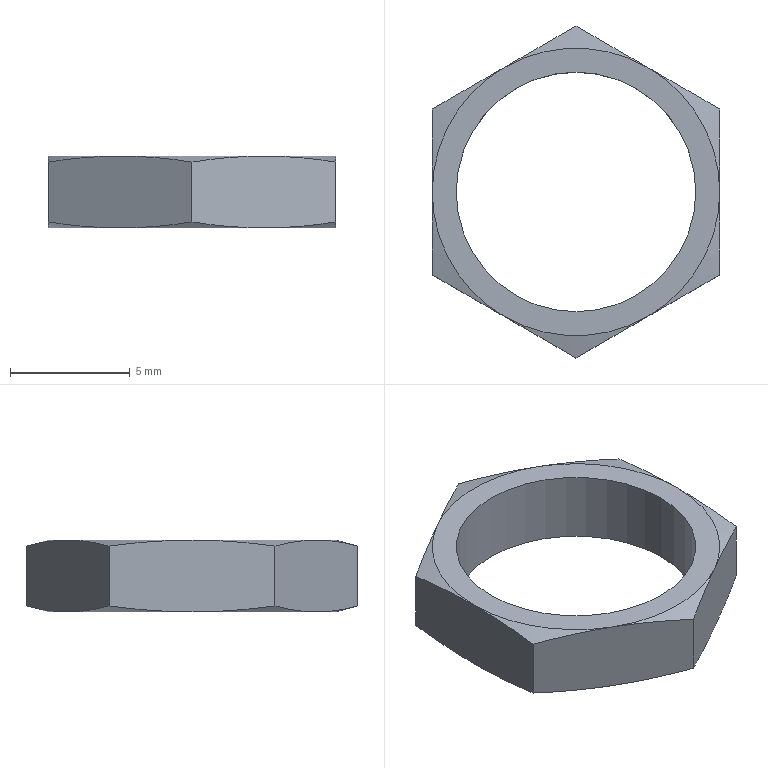Component | SolidWorks | gbgbCJPB6-5-B(0)F8-1_gbgbSNPS-006_CJPF8-2 | 1 solid | 22 faces | box 12 x 13.86 x 3 mm | volume 137 mm3 | cone 12 | plane 8 | cylinder 2 | commonest cylinder face diameters 10 x2
STEP:
#1=COLOUR_RGB('',0.7922,0.8196,0.9333);
#2=FILL_AREA_STYLE_COLOUR('',#1);
#3=FILL_AREA_STYLE('',(#2));
#4=SURFACE_STYLE_FILL_AREA(#3);
#5=SURFACE_SIDE_STYLE('',(#4));
#6=SURFACE_STYLE_USAGE(.BOTH.,#5);
#7=PRESENTATION_STYLE_ASSIGNMENT((#6));
#8=CARTESIAN_POINT('',(2.212,14.172,15.836));
#9=VERTEX_POINT('',#8);
#10=CARTESIAN_POINT('',(2.606,14.172,15.836));
#11=VERTEX_POINT('',#10);
#12=CARTESIAN_POINT('',(2.409,14.172,15.836));
#13=DIRECTION('',(0.,0.,1.));
#14=DIRECTION('',(-1.,0.,0.));
#15=AXIS2_PLACEMENT_3D('',#12,#13,#14);
#16=CIRCLE('',#15,0.1969);
#17=EDGE_CURVE('',#9,#11,#16,.T.);
#18=ORIENTED_EDGE('',*,*,#17,.F.);
#19=CARTESIAN_POINT('',(2.212,14.172,15.954));
#20=VERTEX_POINT('',#19);
#21=CARTESIAN_POINT('',(2.212,14.172,15.836));
#22=DIRECTION('',(0.,0.,1.));
#23=VECTOR('',#22,39.37);
#24=LINE('',#21,#23);
#25=EDGE_CURVE('',#9,#20,#24,.T.);
#26=ORIENTED_EDGE('',*,*,#25,.T.);
#27=CARTESIAN_POINT('',(2.606,14.172,15.954));
#28=VERTEX_POINT('',#27);
#29=CARTESIAN_POINT('',(2.409,14.172,15.954));
#30=DIRECTION('',(0.,0.,1.));
#31=DIRECTION('',(1.,0.,0.));
#32=AXIS2_PLACEMENT_3D('',#29,#30,#31);
#33=CIRCLE('',#32,0.1969);
#34=EDGE_CURVE('',#20,#28,#33,.T.);
#35=ORIENTED_EDGE('',*,*,#34,.T.);
#36=CARTESIAN_POINT('',(2.606,14.172,15.836));
#37=DIRECTION('',(0.,0.,1.));
#38=VECTOR('',#37,39.37);
#39=LINE('',#36,#38);
#40=EDGE_CURVE('',#11,#28,#39,.T.);
#41=ORIENTED_EDGE('',*,*,#40,.F.);
#42=EDGE_LOOP('',(#18,#26,#35,#41));
#43=FACE_OUTER_BOUND('',#42,.T.);
#44=CARTESIAN_POINT('',(2.409,14.172,15.836));
#45=DIRECTION('',(0.,0.,1.));
#46=DIRECTION('',(1.,0.,0.));
#47=AXIS2_PLACEMENT_3D('',#44,#45,#46);
#48=CYLINDRICAL_SURFACE('',#47,0.1969);
#49=ADVANCED_FACE('',(#43),#48,.F.);
#50=CARTESIAN_POINT('',(2.291,14.377,15.836));
#51=VERTEX_POINT('',#50);
#52=CARTESIAN_POINT('',(2.409,14.445,15.846));
#53=VERTEX_POINT('',#52);
#54=CARTESIAN_POINT('',(2.291,14.377,15.836));
#55=CARTESIAN_POINT('',(2.331,14.399,15.836));
#56=CARTESIAN_POINT('',(2.37,14.422,15.84));
#57=CARTESIAN_POINT('',(2.409,14.445,15.846));
#58=B_SPLINE_CURVE_WITH_KNOTS('',3,(#54,#55,#56,#57),.UNSPECIFIED.,.F.,.F.,(4,4),(0.003464,0.006928),.UNSPECIFIED.);
#59=EDGE_CURVE('',#51,#53,#58,.T.);
#60=ORIENTED_EDGE('',*,*,#59,.T.);
#61=CARTESIAN_POINT('',(2.527,14.377,15.836));
#62=VERTEX_POINT('',#61);
#63=CARTESIAN_POINT('',(2.409,14.445,15.846));
#64=CARTESIAN_POINT('',(2.449,14.422,15.84));
#65=CARTESIAN_POINT('',(2.488,14.399,15.836));
#66=CARTESIAN_POINT('',(2.527,14.377,15.836));
#67=B_SPLINE_CURVE_WITH_KNOTS('',3,(#63,#64,#65,#66),.UNSPECIFIED.,.F.,.F.,(4,4),(0.00000023,0.003464),.UNSPECIFIED.);
#68=EDGE_CURVE('',#53,#62,#67,.T.);
#69=ORIENTED_EDGE('',*,*,#68,.T.);
#70=CARTESIAN_POINT('',(2.409,14.172,15.836));
#71=DIRECTION('',(0.,0.,1.));
#72=DIRECTION('',(1.,0.,0.));
#73=AXIS2_PLACEMENT_3D('',#70,#71,#72);
#74=CIRCLE('',#73,0.2362);
#75=EDGE_CURVE('',#62,#51,#74,.T.);
#76=ORIENTED_EDGE('',*,*,#75,.T.);
#77=EDGE_LOOP('',(#60,#69,#76));
#78=FACE_OUTER_BOUND('',#77,.T.);
#79=CARTESIAN_POINT('',(2.409,14.172,15.836));
#80=DIRECTION('',(0.,0.,1.));
#81=DIRECTION('',(1.,0.,0.));
#82=AXIS2_PLACEMENT_3D('',#79,#80,#81);
#83=CONICAL_SURFACE('',#82,0.2362,1.309);
#84=ADVANCED_FACE('',(#78),#83,.T.);
#85=CARTESIAN_POINT('',(2.645,14.172,15.836));
#86=VERTEX_POINT('',#85);
#87=CARTESIAN_POINT('',(2.409,14.172,15.836));
#88=DIRECTION('',(0.,0.,1.));
#89=DIRECTION('',(1.,0.,0.));
#90=AXIS2_PLACEMENT_3D('',#87,#88,#89);
#91=CIRCLE('',#90,0.2362);
#92=EDGE_CURVE('',#86,#62,#91,.T.);
#93=ORIENTED_EDGE('',*,*,#92,.T.);
#94=CARTESIAN_POINT('',(2.645,14.308,15.846));
#95=VERTEX_POINT('',#94);
#96=CARTESIAN_POINT('',(2.527,14.377,15.836));
#97=CARTESIAN_POINT('',(2.567,14.354,15.836));
#98=CARTESIAN_POINT('',(2.606,14.331,15.84));
#99=CARTESIAN_POINT('',(2.645,14.308,15.846));
#100=B_SPLINE_CURVE_WITH_KNOTS('',3,(#96,#97,#98,#99),.UNSPECIFIED.,.F.,.F.,(4,4),(0.003464,0.006928),.UNSPECIFIED.);
#101=EDGE_CURVE('',#62,#95,#100,.T.);
#102=ORIENTED_EDGE('',*,*,#101,.T.);
#103=CARTESIAN_POINT('',(2.645,14.308,15.846));
#104=CARTESIAN_POINT('',(2.645,14.263,15.84));
#105=CARTESIAN_POINT('',(2.645,14.218,15.836));
#106=CARTESIAN_POINT('',(2.645,14.172,15.836));
#107=B_SPLINE_CURVE_WITH_KNOTS('',3,(#103,#104,#105,#106),.UNSPECIFIED.,.F.,.F.,(4,4),(0.01347,0.01695),.UNSPECIFIED.);
#108=EDGE_CURVE('',#95,#86,#107,.T.);
#109=ORIENTED_EDGE('',*,*,#108,.T.);
#110=EDGE_LOOP('',(#93,#102,#109));
#111=FACE_OUTER_BOUND('',#110,.T.);
#112=CARTESIAN_POINT('',(2.409,14.172,15.836));
#113=DIRECTION('',(0.,0.,1.));
#114=DIRECTION('',(1.,0.,0.));
#115=AXIS2_PLACEMENT_3D('',#112,#113,#114);
#116=CONICAL_SURFACE('',#115,0.2362,1.309);
#117=ADVANCED_FACE('',(#111),#116,.T.);
#118=CARTESIAN_POINT('',(2.527,13.967,15.836));
#119=VERTEX_POINT('',#118);
#120=CARTESIAN_POINT('',(2.409,14.172,15.836));
#121=DIRECTION('',(0.,0.,1.));
#122=DIRECTION('',(1.,0.,0.));
#123=AXIS2_PLACEMENT_3D('',#120,#121,#122);
#124=CIRCLE('',#123,0.2362);
#125=EDGE_CURVE('',#119,#86,#124,.T.);
#126=ORIENTED_EDGE('',*,*,#125,.T.);
#127=CARTESIAN_POINT('',(2.645,14.036,15.846));
#128=VERTEX_POINT('',#127);
#129=CARTESIAN_POINT('',(2.645,14.172,15.836));
#130=CARTESIAN_POINT('',(2.645,14.149,15.836));
#131=CARTESIAN_POINT('',(2.645,14.127,15.837));
#132=CARTESIAN_POINT('',(2.645,14.081,15.84));
#133=CARTESIAN_POINT('',(2.645,14.058,15.843));
#134=CARTESIAN_POINT('',(2.645,14.036,15.846));
#135=B_SPLINE_CURVE_WITH_KNOTS('',3,(#129,#130,#131,#132,#133,#134),.UNSPECIFIED.,.F.,.F.,(4,2,4),(0.01695,0.01869,0.02043),.UNSPECIFIED.);
#136=EDGE_CURVE('',#86,#128,#135,.T.);
#137=ORIENTED_EDGE('',*,*,#136,.T.);
#138=CARTESIAN_POINT('',(2.645,14.036,15.846));
#139=CARTESIAN_POINT('',(2.606,14.013,15.84));
#140=CARTESIAN_POINT('',(2.567,13.99,15.836));
#141=CARTESIAN_POINT('',(2.527,13.967,15.836));
#142=B_SPLINE_CURVE_WITH_KNOTS('',3,(#138,#139,#140,#141),.UNSPECIFIED.,.F.,.F.,(4,4),(0.00000023,0.003464),.UNSPECIFIED.);
#143=EDGE_CURVE('',#128,#119,#142,.T.);
#144=ORIENTED_EDGE('',*,*,#143,.T.);
#145=EDGE_LOOP('',(#126,#137,#144));
#146=FACE_OUTER_BOUND('',#145,.T.);
#147=CARTESIAN_POINT('',(2.409,14.172,15.836));
#148=DIRECTION('',(0.,0.,1.));
#149=DIRECTION('',(1.,0.,0.));
#150=AXIS2_PLACEMENT_3D('',#147,#148,#149);
#151=CONICAL_SURFACE('',#150,0.2362,1.309);
#152=ADVANCED_FACE('',(#146),#151,.T.);
#153=CARTESIAN_POINT('',(2.291,13.967,15.836));
#154=VERTEX_POINT('',#153);
#155=CARTESIAN_POINT('',(2.409,14.172,15.836));
#156=DIRECTION('',(0.,0.,1.));
#157=DIRECTION('',(1.,0.,0.));
#158=AXIS2_PLACEMENT_3D('',#155,#156,#157);
#159=CIRCLE('',#158,0.2362);
#160=EDGE_CURVE('',#154,#119,#159,.T.);
#161=ORIENTED_EDGE('',*,*,#160,.T.);
#162=CARTESIAN_POINT('',(2.409,13.899,15.846));
#163=VERTEX_POINT('',#162);
#164=CARTESIAN_POINT('',(2.527,13.967,15.836));
#165=CARTESIAN_POINT('',(2.488,13.945,15.836));
#166=CARTESIAN_POINT('',(2.449,13.922,15.84));
#167=CARTESIAN_POINT('',(2.409,13.899,15.846));
#168=B_SPLINE_CURVE_WITH_KNOTS('',3,(#164,#165,#166,#167),.UNSPECIFIED.,.F.,.F.,(4,4),(0.003464,0.006928),.UNSPECIFIED.);
#169=EDGE_CURVE('',#119,#163,#168,.T.);
#170=ORIENTED_EDGE('',*,*,#169,.T.);
#171=CARTESIAN_POINT('',(2.409,13.899,15.846));
#172=CARTESIAN_POINT('',(2.37,13.922,15.84));
#173=CARTESIAN_POINT('',(2.331,13.945,15.836));
#174=CARTESIAN_POINT('',(2.291,13.967,15.836));
#175=B_SPLINE_CURVE_WITH_KNOTS('',3,(#171,#172,#173,#174),.UNSPECIFIED.,.F.,.F.,(4,4),(0.00000023,0.003464),.UNSPECIFIED.);
#176=EDGE_CURVE('',#163,#154,#175,.T.);
#177=ORIENTED_EDGE('',*,*,#176,.T.);
#178=EDGE_LOOP('',(#161,#170,#177));
#179=FACE_OUTER_BOUND('',#178,.T.);
#180=CARTESIAN_POINT('',(2.409,14.172,15.836));
#181=DIRECTION('',(0.,0.,1.));
#182=DIRECTION('',(1.,0.,0.));
#183=AXIS2_PLACEMENT_3D('',#180,#181,#182);
#184=CONICAL_SURFACE('',#183,0.2362,1.309);
#185=ADVANCED_FACE('',(#179),#184,.T.);
#186=CARTESIAN_POINT('',(2.173,14.172,15.836));
#187=VERTEX_POINT('',#186);
#188=CARTESIAN_POINT('',(2.409,14.172,15.836));
#189=DIRECTION('',(0.,0.,1.));
#190=DIRECTION('',(1.,0.,0.));
#191=AXIS2_PLACEMENT_3D('',#188,#189,#190);
#192=CIRCLE('',#191,0.2362);
#193=EDGE_CURVE('',#187,#154,#192,.T.);
#194=ORIENTED_EDGE('',*,*,#193,.T.);
#195=CARTESIAN_POINT('',(2.173,14.036,15.846));
#196=VERTEX_POINT('',#195);
#197=CARTESIAN_POINT('',(2.291,13.967,15.836));
#198=CARTESIAN_POINT('',(2.252,13.99,15.836));
#199=CARTESIAN_POINT('',(2.212,14.013,15.84));
#200=CARTESIAN_POINT('',(2.173,14.036,15.846));
#201=B_SPLINE_CURVE_WITH_KNOTS('',3,(#197,#198,#199,#200),.UNSPECIFIED.,.F.,.F.,(4,4),(0.003464,0.006928),.UNSPECIFIED.);
#202=EDGE_CURVE('',#154,#196,#201,.T.);
#203=ORIENTED_EDGE('',*,*,#202,.T.);
#204=CARTESIAN_POINT('',(2.173,14.036,15.846));
#205=CARTESIAN_POINT('',(2.173,14.058,15.843));
#206=CARTESIAN_POINT('',(2.173,14.081,15.84));
#207=CARTESIAN_POINT('',(2.173,14.127,15.837));
#208=CARTESIAN_POINT('',(2.173,14.149,15.836));
#209=CARTESIAN_POINT('',(2.173,14.172,15.836));
#210=B_SPLINE_CURVE_WITH_KNOTS('',3,(#204,#205,#206,#207,#208,#209),.UNSPECIFIED.,.F.,.F.,(4,2,4),(0.005848,0.007589,0.009329),.UNSPECIFIED.);
#211=EDGE_CURVE('',#196,#187,#210,.T.);
#212=ORIENTED_EDGE('',*,*,#211,.T.);
#213=EDGE_LOOP('',(#194,#203,#212));
#214=FACE_OUTER_BOUND('',#213,.T.);
#215=CARTESIAN_POINT('',(2.409,14.172,15.836));
#216=DIRECTION('',(0.,0.,1.));
#217=DIRECTION('',(1.,0.,0.));
#218=AXIS2_PLACEMENT_3D('',#215,#216,#217);
#219=CONICAL_SURFACE('',#218,0.2362,1.309);
#220=ADVANCED_FACE('',(#214),#219,.T.);
#221=CARTESIAN_POINT('',(2.291,13.967,15.954));
#222=VERTEX_POINT('',#221);
#223=CARTESIAN_POINT('',(2.409,13.899,15.944));
#224=VERTEX_POINT('',#223);
#225=CARTESIAN_POINT('',(2.291,13.967,15.954));
#226=CARTESIAN_POINT('',(2.331,13.945,15.954));
#227=CARTESIAN_POINT('',(2.37,13.922,15.95));
#228=CARTESIAN_POINT('',(2.409,13.899,15.944));
#229=B_SPLINE_CURVE_WITH_KNOTS('',3,(#225,#226,#227,#228),.UNSPECIFIED.,.F.,.F.,(4,4),(0.003464,0.006928),.UNSPECIFIED.);
#230=EDGE_CURVE('',#222,#224,#229,.T.);
#231=ORIENTED_EDGE('',*,*,#230,.T.);
#232=CARTESIAN_POINT('',(2.527,13.967,15.954));
#233=VERTEX_POINT('',#232);
#234=CARTESIAN_POINT('',(2.409,13.899,15.944));
#235=CARTESIAN_POINT('',(2.449,13.922,15.95));
#236=CARTESIAN_POINT('',(2.488,13.945,15.954));
#237=CARTESIAN_POINT('',(2.527,13.967,15.954));
#238=B_SPLINE_CURVE_WITH_KNOTS('',3,(#234,#235,#236,#237),.UNSPECIFIED.,.F.,.F.,(4,4),(0.00000023,0.003464),.UNSPECIFIED.);
#239=EDGE_CURVE('',#224,#233,#238,.T.);
#240=ORIENTED_EDGE('',*,*,#239,.T.);
#241=CARTESIAN_POINT('',(2.409,14.172,15.954));
#242=DIRECTION('',(0.,0.,1.));
#243=DIRECTION('',(1.,0.,0.));
#244=AXIS2_PLACEMENT_3D('',#241,#242,#243);
#245=CIRCLE('',#244,0.2362);
#246=EDGE_CURVE('',#222,#233,#245,.T.);
#247=ORIENTED_EDGE('',*,*,#246,.F.);
#248=EDGE_LOOP('',(#231,#240,#247));
#249=FACE_OUTER_BOUND('',#248,.T.);
#250=CARTESIAN_POINT('',(2.409,14.172,15.916));
#251=DIRECTION('',(0.,-0.,-1.));
#252=DIRECTION('',(-1.,0.,0.));
#253=AXIS2_PLACEMENT_3D('',#250,#251,#252);
#254=CONICAL_SURFACE('',#253,0.378,1.309);
#255=ADVANCED_FACE('',(#249),#254,.T.);
#256=CARTESIAN_POINT('',(2.645,14.172,15.954));
#257=VERTEX_POINT('',#256);
#258=CARTESIAN_POINT('',(2.409,14.172,15.954));
#259=DIRECTION('',(0.,0.,1.));
#260=DIRECTION('',(1.,0.,0.));
#261=AXIS2_PLACEMENT_3D('',#258,#259,#260);
#262=CIRCLE('',#261,0.2362);
#263=EDGE_CURVE('',#233,#257,#262,.T.);
#264=ORIENTED_EDGE('',*,*,#263,.F.);
#265=CARTESIAN_POINT('',(2.645,14.036,15.944));
#266=VERTEX_POINT('',#265);
#267=CARTESIAN_POINT('',(2.527,13.967,15.954));
#268=CARTESIAN_POINT('',(2.567,13.99,15.954));
#269=CARTESIAN_POINT('',(2.606,14.013,15.95));
#270=CARTESIAN_POINT('',(2.645,14.036,15.944));
#271=B_SPLINE_CURVE_WITH_KNOTS('',3,(#267,#268,#269,#270),.UNSPECIFIED.,.F.,.F.,(4,4),(0.003464,0.006928),.UNSPECIFIED.);
#272=EDGE_CURVE('',#233,#266,#271,.T.);
#273=ORIENTED_EDGE('',*,*,#272,.T.);
#274=CARTESIAN_POINT('',(2.645,14.036,15.944));
#275=CARTESIAN_POINT('',(2.645,14.058,15.947));
#276=CARTESIAN_POINT('',(2.645,14.081,15.95));
#277=CARTESIAN_POINT('',(2.645,14.127,15.953));
#278=CARTESIAN_POINT('',(2.645,14.149,15.954));
#279=CARTESIAN_POINT('',(2.645,14.172,15.954));
#280=B_SPLINE_CURVE_WITH_KNOTS('',3,(#274,#275,#276,#277,#278,#279),.UNSPECIFIED.,.F.,.F.,(4,2,4),(0.005848,0.007589,0.009329),.UNSPECIFIED.);
#281=EDGE_CURVE('',#266,#257,#280,.T.);
#282=ORIENTED_EDGE('',*,*,#281,.T.);
#283=EDGE_LOOP('',(#264,#273,#282));
#284=FACE_OUTER_BOUND('',#283,.T.);
#285=CARTESIAN_POINT('',(2.409,14.172,15.916));
#286=DIRECTION('',(0.,-0.,-1.));
#287=DIRECTION('',(-1.,0.,0.));
#288=AXIS2_PLACEMENT_3D('',#285,#286,#287);
#289=CONICAL_SURFACE('',#288,0.378,1.309);
#290=ADVANCED_FACE('',(#284),#289,.T.);
#291=CARTESIAN_POINT('',(2.527,14.377,15.954));
#292=VERTEX_POINT('',#291);
#293=CARTESIAN_POINT('',(2.409,14.172,15.954));
#294=DIRECTION('',(0.,0.,1.));
#295=DIRECTION('',(1.,0.,0.));
#296=AXIS2_PLACEMENT_3D('',#293,#294,#295);
#297=CIRCLE('',#296,0.2362);
#298=EDGE_CURVE('',#257,#292,#297,.T.);
#299=ORIENTED_EDGE('',*,*,#298,.F.);
#300=CARTESIAN_POINT('',(2.645,14.308,15.944));
#301=VERTEX_POINT('',#300);
#302=CARTESIAN_POINT('',(2.645,14.172,15.954));
#303=CARTESIAN_POINT('',(2.645,14.218,15.954));
#304=CARTESIAN_POINT('',(2.645,14.263,15.95));
#305=CARTESIAN_POINT('',(2.645,14.308,15.944));
#306=B_SPLINE_CURVE_WITH_KNOTS('',3,(#302,#303,#304,#305),.UNSPECIFIED.,.F.,.F.,(4,4),(0.009329,0.01282),.UNSPECIFIED.);
#307=EDGE_CURVE('',#257,#301,#306,.T.);
#308=ORIENTED_EDGE('',*,*,#307,.T.);
#309=CARTESIAN_POINT('',(2.645,14.308,15.944));
#310=CARTESIAN_POINT('',(2.606,14.331,15.95));
#311=CARTESIAN_POINT('',(2.567,14.354,15.954));
#312=CARTESIAN_POINT('',(2.527,14.377,15.954));
#313=B_SPLINE_CURVE_WITH_KNOTS('',3,(#309,#310,#311,#312),.UNSPECIFIED.,.F.,.F.,(4,4),(0.00000023,0.003464),.UNSPECIFIED.);
#314=EDGE_CURVE('',#301,#292,#313,.T.);
#315=ORIENTED_EDGE('',*,*,#314,.T.);
#316=EDGE_LOOP('',(#299,#308,#315));
#317=FACE_OUTER_BOUND('',#316,.T.);
#318=CARTESIAN_POINT('',(2.409,14.172,15.916));
#319=DIRECTION('',(0.,-0.,-1.));
#320=DIRECTION('',(-1.,0.,0.));
#321=AXIS2_PLACEMENT_3D('',#318,#319,#320);
#322=CONICAL_SURFACE('',#321,0.378,1.309);
#323=ADVANCED_FACE('',(#317),#322,.T.);
#324=CARTESIAN_POINT('',(2.173,14.172,15.954));
#325=VERTEX_POINT('',#324);
#326=CARTESIAN_POINT('',(2.173,14.036,15.944));
#327=VERTEX_POINT('',#326);
#328=CARTESIAN_POINT('',(2.173,14.172,15.954));
#329=CARTESIAN_POINT('',(2.173,14.149,15.954));
#330=CARTESIAN_POINT('',(2.173,14.127,15.953));
#331=CARTESIAN_POINT('',(2.173,14.081,15.95));
#332=CARTESIAN_POINT('',(2.173,14.058,15.947));
#333=CARTESIAN_POINT('',(2.173,14.036,15.944));
#334=B_SPLINE_CURVE_WITH_KNOTS('',3,(#328,#329,#330,#331,#332,#333),.UNSPECIFIED.,.F.,.F.,(4,2,4),(0.01695,0.01869,0.02043),.UNSPECIFIED.);
#335=EDGE_CURVE('',#325,#327,#334,.T.);
#336=ORIENTED_EDGE('',*,*,#335,.T.);
#337=CARTESIAN_POINT('',(2.173,14.036,15.944));
#338=CARTESIAN_POINT('',(2.212,14.013,15.95));
#339=CARTESIAN_POINT('',(2.252,13.99,15.954));
#340=CARTESIAN_POINT('',(2.291,13.967,15.954));
#341=B_SPLINE_CURVE_WITH_KNOTS('',3,(#337,#338,#339,#340),.UNSPECIFIED.,.F.,.F.,(4,4),(0.00000023,0.003464),.UNSPECIFIED.);
#342=EDGE_CURVE('',#327,#222,#341,.T.);
#343=ORIENTED_EDGE('',*,*,#342,.T.);
#344=CARTESIAN_POINT('',(2.409,14.172,15.954));
#345=DIRECTION('',(0.,0.,1.));
#346=DIRECTION('',(1.,0.,0.));
#347=AXIS2_PLACEMENT_3D('',#344,#345,#346);
#348=CIRCLE('',#347,0.2362);
#349=EDGE_CURVE('',#325,#222,#348,.T.);
#350=ORIENTED_EDGE('',*,*,#349,.F.);
#351=EDGE_LOOP('',(#336,#343,#350));
#352=FACE_OUTER_BOUND('',#351,.T.);
#353=CARTESIAN_POINT('',(2.409,14.172,15.916));
#354=DIRECTION('',(0.,-0.,-1.));
#355=DIRECTION('',(-1.,0.,0.));
#356=AXIS2_PLACEMENT_3D('',#353,#354,#355);
#357=CONICAL_SURFACE('',#356,0.378,1.309);
#358=ADVANCED_FACE('',(#352),#357,.T.);
#359=CARTESIAN_POINT('',(2.291,14.377,15.954));
#360=VERTEX_POINT('',#359);
#361=CARTESIAN_POINT('',(2.409,14.172,15.954));
#362=DIRECTION('',(0.,0.,1.));
#363=DIRECTION('',(1.,0.,0.));
#364=AXIS2_PLACEMENT_3D('',#361,#362,#363);
#365=CIRCLE('',#364,0.2362);
#366=EDGE_CURVE('',#292,#360,#365,.T.);
#367=ORIENTED_EDGE('',*,*,#366,.F.);
#368=CARTESIAN_POINT('',(2.409,14.445,15.944));
#369=VERTEX_POINT('',#368);
#370=CARTESIAN_POINT('',(2.527,14.377,15.954));
#371=CARTESIAN_POINT('',(2.488,14.399,15.954));
#372=CARTESIAN_POINT('',(2.449,14.422,15.95));
#373=CARTESIAN_POINT('',(2.409,14.445,15.944));
#374=B_SPLINE_CURVE_WITH_KNOTS('',3,(#370,#371,#372,#373),.UNSPECIFIED.,.F.,.F.,(4,4),(0.003464,0.006928),.UNSPECIFIED.);
#375=EDGE_CURVE('',#292,#369,#374,.T.);
#376=ORIENTED_EDGE('',*,*,#375,.T.);
#377=CARTESIAN_POINT('',(2.409,14.445,15.944));
#378=CARTESIAN_POINT('',(2.37,14.422,15.95));
#379=CARTESIAN_POINT('',(2.331,14.399,15.954));
#380=CARTESIAN_POINT('',(2.291,14.377,15.954));
#381=B_SPLINE_CURVE_WITH_KNOTS('',3,(#377,#378,#379,#380),.UNSPECIFIED.,.F.,.F.,(4,4),(0.00000023,0.003464),.UNSPECIFIED.);
#382=EDGE_CURVE('',#369,#360,#381,.T.);
#383=ORIENTED_EDGE('',*,*,#382,.T.);
#384=EDGE_LOOP('',(#367,#376,#383));
#385=FACE_OUTER_BOUND('',#384,.T.);
#386=CARTESIAN_POINT('',(2.409,14.172,15.916));
#387=DIRECTION('',(0.,-0.,-1.));
#388=DIRECTION('',(-1.,0.,0.));
#389=AXIS2_PLACEMENT_3D('',#386,#387,#388);
#390=CONICAL_SURFACE('',#389,0.378,1.309);
#391=ADVANCED_FACE('',(#385),#390,.T.);
#392=CARTESIAN_POINT('',(2.409,14.172,15.954));
#393=DIRECTION('',(0.,0.,1.));
#394=DIRECTION('',(1.,0.,0.));
#395=AXIS2_PLACEMENT_3D('',#392,#393,#394);
#396=CIRCLE('',#395,0.1969);
#397=EDGE_CURVE('',#28,#20,#396,.T.);
#398=ORIENTED_EDGE('',*,*,#397,.F.);
#399=ORIENTED_EDGE('',*,*,#34,.F.);
#400=EDGE_LOOP('',(#398,#399));
#401=FACE_BOUND('',#400,.T.);
#402=ORIENTED_EDGE('',*,*,#298,.T.);
#403=ORIENTED_EDGE('',*,*,#366,.T.);
#404=CARTESIAN_POINT('',(2.409,14.172,15.954));
#405=DIRECTION('',(0.,0.,1.));
#406=DIRECTION('',(1.,0.,0.));
#407=AXIS2_PLACEMENT_3D('',#404,#405,#406);
#408=CIRCLE('',#407,0.2362);
#409=EDGE_CURVE('',#360,#325,#408,.T.);
#410=ORIENTED_EDGE('',*,*,#409,.T.);
#411=ORIENTED_EDGE('',*,*,#349,.T.);
#412=ORIENTED_EDGE('',*,*,#246,.T.);
#413=ORIENTED_EDGE('',*,*,#263,.T.);
#414=EDGE_LOOP('',(#402,#403,#410,#411,#412,#413));
#415=FACE_OUTER_BOUND('',#414,.T.);
#416=CARTESIAN_POINT('',(2.409,14.408,15.954));
#417=DIRECTION('',(0.,-0.,-1.));
#418=DIRECTION('',(-1.,0.,-0.));
#419=AXIS2_PLACEMENT_3D('',#416,#417,#418);
#420=PLANE('',#419);
#421=ADVANCED_FACE('',(#401,#415),#420,.F.);
#422=ORIENTED_EDGE('',*,*,#25,.F.);
#423=CARTESIAN_POINT('',(2.409,14.172,15.836));
#424=DIRECTION('',(0.,0.,1.));
#425=DIRECTION('',(-1.,0.,0.));
#426=AXIS2_PLACEMENT_3D('',#423,#424,#425);
#427=CIRCLE('',#426,0.1969);
#428=EDGE_CURVE('',#11,#9,#427,.T.);
#429=ORIENTED_EDGE('',*,*,#428,.F.);
#430=ORIENTED_EDGE('',*,*,#40,.T.);
#431=ORIENTED_EDGE('',*,*,#397,.T.);
#432=EDGE_LOOP('',(#422,#429,#430,#431));
#433=FACE_OUTER_BOUND('',#432,.T.);
#434=CARTESIAN_POINT('',(2.409,14.172,15.836));
#435=DIRECTION('',(0.,0.,1.));
#436=DIRECTION('',(1.,0.,0.));
#437=AXIS2_PLACEMENT_3D('',#434,#435,#436);
#438=CYLINDRICAL_SURFACE('',#437,0.1969);
#439=ADVANCED_FACE('',(#433),#438,.F.);
#440=ORIENTED_EDGE('',*,*,#92,.F.);
#441=ORIENTED_EDGE('',*,*,#125,.F.);
#442=ORIENTED_EDGE('',*,*,#160,.F.);
#443=ORIENTED_EDGE('',*,*,#193,.F.);
#444=CARTESIAN_POINT('',(2.409,14.172,15.836));
#445=DIRECTION('',(0.,0.,1.));
#446=DIRECTION('',(1.,0.,0.));
#447=AXIS2_PLACEMENT_3D('',#444,#445,#446);
#448=CIRCLE('',#447,0.2362);
#449=EDGE_CURVE('',#51,#187,#448,.T.);
#450=ORIENTED_EDGE('',*,*,#449,.F.);
#451=ORIENTED_EDGE('',*,*,#75,.F.);
#452=EDGE_LOOP('',(#440,#441,#442,#443,#450,#451));
#453=FACE_OUTER_BOUND('',#452,.T.);
#454=ORIENTED_EDGE('',*,*,#428,.T.);
#455=ORIENTED_EDGE('',*,*,#17,.T.);
#456=EDGE_LOOP('',(#454,#455));
#457=FACE_BOUND('',#456,.T.);
#458=CARTESIAN_POINT('',(2.409,14.369,15.836));
#459=DIRECTION('',(0.,0.,1.));
#460=DIRECTION('',(1.,-0.,0.));
#461=AXIS2_PLACEMENT_3D('',#458,#459,#460);
#462=PLANE('',#461);
#463=ADVANCED_FACE('',(#453,#457),#462,.F.);
#464=ORIENTED_EDGE('',*,*,#449,.T.);
#465=CARTESIAN_POINT('',(2.173,14.308,15.846));
#466=VERTEX_POINT('',#465);
#467=CARTESIAN_POINT('',(2.173,14.172,15.836));
#468=CARTESIAN_POINT('',(2.173,14.218,15.836));
#469=CARTESIAN_POINT('',(2.173,14.263,15.84));
#470=CARTESIAN_POINT('',(2.173,14.308,15.846));
#471=B_SPLINE_CURVE_WITH_KNOTS('',3,(#467,#468,#469,#470),.UNSPECIFIED.,.F.,.F.,(4,4),(0.009329,0.01282),.UNSPECIFIED.);
#472=EDGE_CURVE('',#187,#466,#471,.T.);
#473=ORIENTED_EDGE('',*,*,#472,.T.);
#474=CARTESIAN_POINT('',(2.173,14.308,15.846));
#475=CARTESIAN_POINT('',(2.212,14.331,15.84));
#476=CARTESIAN_POINT('',(2.252,14.354,15.836));
#477=CARTESIAN_POINT('',(2.291,14.377,15.836));
#478=B_SPLINE_CURVE_WITH_KNOTS('',3,(#474,#475,#476,#477),.UNSPECIFIED.,.F.,.F.,(4,4),(0.00000023,0.003464),.UNSPECIFIED.);
#479=EDGE_CURVE('',#466,#51,#478,.T.);
#480=ORIENTED_EDGE('',*,*,#479,.T.);
#481=EDGE_LOOP('',(#464,#473,#480));
#482=FACE_OUTER_BOUND('',#481,.T.);
#483=CARTESIAN_POINT('',(2.409,14.172,15.836));
#484=DIRECTION('',(0.,0.,1.));
#485=DIRECTION('',(1.,0.,0.));
#486=AXIS2_PLACEMENT_3D('',#483,#484,#485);
#487=CONICAL_SURFACE('',#486,0.2362,1.309);
#488=ADVANCED_FACE('',(#482),#487,.T.);
#489=CARTESIAN_POINT('',(2.173,14.308,15.944));
#490=VERTEX_POINT('',#489);
#491=CARTESIAN_POINT('',(2.291,14.377,15.954));
#492=CARTESIAN_POINT('',(2.252,14.354,15.954));
#493=CARTESIAN_POINT('',(2.212,14.331,15.95));
#494=CARTESIAN_POINT('',(2.173,14.308,15.944));
#495=B_SPLINE_CURVE_WITH_KNOTS('',3,(#491,#492,#493,#494),.UNSPECIFIED.,.F.,.F.,(4,4),(0.003464,0.006928),.UNSPECIFIED.);
#496=EDGE_CURVE('',#360,#490,#495,.T.);
#497=ORIENTED_EDGE('',*,*,#496,.T.);
#498=CARTESIAN_POINT('',(2.173,14.308,15.944));
#499=CARTESIAN_POINT('',(2.173,14.263,15.95));
#500=CARTESIAN_POINT('',(2.173,14.218,15.954));
#501=CARTESIAN_POINT('',(2.173,14.172,15.954));
#502=B_SPLINE_CURVE_WITH_KNOTS('',3,(#498,#499,#500,#501),.UNSPECIFIED.,.F.,.F.,(4,4),(0.01347,0.01695),.UNSPECIFIED.);
#503=EDGE_CURVE('',#490,#325,#502,.T.);
#504=ORIENTED_EDGE('',*,*,#503,.T.);
#505=ORIENTED_EDGE('',*,*,#409,.F.);
#506=EDGE_LOOP('',(#497,#504,#505));
#507=FACE_OUTER_BOUND('',#506,.T.);
#508=CARTESIAN_POINT('',(2.409,14.172,15.916));
#509=DIRECTION('',(0.,-0.,-1.));
#510=DIRECTION('',(-1.,0.,0.));
#511=AXIS2_PLACEMENT_3D('',#508,#509,#510);
#512=CONICAL_SURFACE('',#511,0.378,1.309);
#513=ADVANCED_FACE('',(#507),#512,.T.);
#514=CARTESIAN_POINT('',(2.409,14.445,15.836));
#515=DIRECTION('',(0.,0.,1.));
#516=VECTOR('',#515,39.37);
#517=LINE('',#514,#516);
#518=EDGE_CURVE('',#53,#369,#517,.T.);
#519=ORIENTED_EDGE('',*,*,#518,.T.);
#520=ORIENTED_EDGE('',*,*,#375,.F.);
#521=ORIENTED_EDGE('',*,*,#314,.F.);
#522=CARTESIAN_POINT('',(2.645,14.308,15.836));
#523=DIRECTION('',(0.,0.,1.));
#524=VECTOR('',#523,39.37);
#525=LINE('',#522,#524);
#526=EDGE_CURVE('',#95,#301,#525,.T.);
#527=ORIENTED_EDGE('',*,*,#526,.F.);
#528=ORIENTED_EDGE('',*,*,#101,.F.);
#529=ORIENTED_EDGE('',*,*,#68,.F.);
#530=EDGE_LOOP('',(#519,#520,#521,#527,#528,#529));
#531=FACE_OUTER_BOUND('',#530,.T.);
#532=CARTESIAN_POINT('',(2.409,14.445,15.836));
#533=DIRECTION('',(-0.5,-0.866,0.));
#534=DIRECTION('',(-0.866,0.5,-0.));
#535=AXIS2_PLACEMENT_3D('',#532,#533,#534);
#536=PLANE('',#535);
#537=ADVANCED_FACE('',(#531),#536,.F.);
#538=ORIENTED_EDGE('',*,*,#526,.T.);
#539=ORIENTED_EDGE('',*,*,#307,.F.);
#540=ORIENTED_EDGE('',*,*,#281,.F.);
#541=CARTESIAN_POINT('',(2.645,14.036,15.836));
#542=DIRECTION('',(0.,0.,1.));
#543=VECTOR('',#542,39.37);
#544=LINE('',#541,#543);
#545=EDGE_CURVE('',#128,#266,#544,.T.);
#546=ORIENTED_EDGE('',*,*,#545,.F.);
#547=ORIENTED_EDGE('',*,*,#136,.F.);
#548=ORIENTED_EDGE('',*,*,#108,.F.);
#549=EDGE_LOOP('',(#538,#539,#540,#546,#547,#548));
#550=FACE_OUTER_BOUND('',#549,.T.);
#551=CARTESIAN_POINT('',(2.645,14.308,15.836));
#552=DIRECTION('',(-1.,0.,-0.));
#553=DIRECTION('',(0.,0.,1.));
#554=AXIS2_PLACEMENT_3D('',#551,#552,#553);
#555=PLANE('',#554);
#556=ADVANCED_FACE('',(#550),#555,.F.);
#557=ORIENTED_EDGE('',*,*,#545,.T.);
#558=ORIENTED_EDGE('',*,*,#272,.F.);
#559=ORIENTED_EDGE('',*,*,#239,.F.);
#560=CARTESIAN_POINT('',(2.409,13.899,15.836));
#561=DIRECTION('',(0.,0.,1.));
#562=VECTOR('',#561,39.37);
#563=LINE('',#560,#562);
#564=EDGE_CURVE('',#163,#224,#563,.T.);
#565=ORIENTED_EDGE('',*,*,#564,.F.);
#566=ORIENTED_EDGE('',*,*,#169,.F.);
#567=ORIENTED_EDGE('',*,*,#143,.F.);
#568=EDGE_LOOP('',(#557,#558,#559,#565,#566,#567));
#569=FACE_OUTER_BOUND('',#568,.T.);
#570=CARTESIAN_POINT('',(2.645,14.036,15.836));
#571=DIRECTION('',(-0.5,0.866,-0.));
#572=DIRECTION('',(0.866,0.5,-0.));
#573=AXIS2_PLACEMENT_3D('',#570,#571,#572);
#574=PLANE('',#573);
#575=ADVANCED_FACE('',(#569),#574,.F.);
#576=ORIENTED_EDGE('',*,*,#564,.T.);
#577=ORIENTED_EDGE('',*,*,#230,.F.);
#578=ORIENTED_EDGE('',*,*,#342,.F.);
#579=CARTESIAN_POINT('',(2.173,14.036,15.836));
#580=DIRECTION('',(0.,0.,1.));
#581=VECTOR('',#580,39.37);
#582=LINE('',#579,#581);
#583=EDGE_CURVE('',#196,#327,#582,.T.);
#584=ORIENTED_EDGE('',*,*,#583,.F.);
#585=ORIENTED_EDGE('',*,*,#202,.F.);
#586=ORIENTED_EDGE('',*,*,#176,.F.);
#587=EDGE_LOOP('',(#576,#577,#578,#584,#585,#586));
#588=FACE_OUTER_BOUND('',#587,.T.);
#589=CARTESIAN_POINT('',(2.409,13.899,15.836));
#590=DIRECTION('',(0.5,0.866,-0.));
#591=DIRECTION('',(0.866,-0.5,0.));
#592=AXIS2_PLACEMENT_3D('',#589,#590,#591);
#593=PLANE('',#592);
#594=ADVANCED_FACE('',(#588),#593,.F.);
#595=ORIENTED_EDGE('',*,*,#583,.T.);
#596=ORIENTED_EDGE('',*,*,#335,.F.);
#597=ORIENTED_EDGE('',*,*,#503,.F.);
#598=CARTESIAN_POINT('',(2.173,14.308,15.836));
#599=DIRECTION('',(0.,0.,1.));
#600=VECTOR('',#599,39.37);
#601=LINE('',#598,#600);
#602=EDGE_CURVE('',#466,#490,#601,.T.);
#603=ORIENTED_EDGE('',*,*,#602,.F.);
#604=ORIENTED_EDGE('',*,*,#472,.F.);
#605=ORIENTED_EDGE('',*,*,#211,.F.);
#606=EDGE_LOOP('',(#595,#596,#597,#603,#604,#605));
#607=FACE_OUTER_BOUND('',#606,.T.);
#608=CARTESIAN_POINT('',(2.173,14.036,15.836));
#609=DIRECTION('',(1.,-0.,0.));
#610=DIRECTION('',(0.,-0.,-1.));
#611=AXIS2_PLACEMENT_3D('',#608,#609,#610);
#612=PLANE('',#611);
#613=ADVANCED_FACE('',(#607),#612,.F.);
#614=ORIENTED_EDGE('',*,*,#602,.T.);
#615=ORIENTED_EDGE('',*,*,#496,.F.);
#616=ORIENTED_EDGE('',*,*,#382,.F.);
#617=ORIENTED_EDGE('',*,*,#518,.F.);
#618=ORIENTED_EDGE('',*,*,#59,.F.);
#619=ORIENTED_EDGE('',*,*,#479,.F.);
#620=EDGE_LOOP('',(#614,#615,#616,#617,#618,#619));
#621=FACE_OUTER_BOUND('',#620,.T.);
#622=CARTESIAN_POINT('',(2.173,14.308,15.836));
#623=DIRECTION('',(0.5,-0.866,0.));
#624=DIRECTION('',(-0.866,-0.5,0.));
#625=AXIS2_PLACEMENT_3D('',#622,#623,#624);
#626=PLANE('',#625);
#627=ADVANCED_FACE('',(#621),#626,.F.);
#628=CLOSED_SHELL('',(#49,#84,#117,#152,#185,#220,#255,#290,#323,#358,#391,#421,#439,#463,#488,#513,#537,#556,#575,#594,#613,#627));
#629=MANIFOLD_SOLID_BREP('',#628);
#630=STYLED_ITEM('',(#7),#629);
#631=(LENGTH_UNIT()NAMED_UNIT(*)SI_UNIT($,.METRE.));
#632=LENGTH_MEASURE_WITH_UNIT(LENGTH_MEASURE(0.0254),#631);
#633=DIMENSIONAL_EXPONENTS(1.,0.,0.,0.,0.,0.,0.);
#634=(CONVERSION_BASED_UNIT('',#632)LENGTH_UNIT()NAMED_UNIT(#633));
#635=UNCERTAINTY_MEASURE_WITH_UNIT(LENGTH_MEASURE(0.00001),#634,'','');
#636=(NAMED_UNIT(*)PLANE_ANGLE_UNIT()SI_UNIT($,.RADIAN.));
#637=(NAMED_UNIT(*)SI_UNIT($,.STERADIAN.)SOLID_ANGLE_UNIT());
#638=(GEOMETRIC_REPRESENTATION_CONTEXT(3)GLOBAL_UNCERTAINTY_ASSIGNED_CONTEXT((#635))GLOBAL_UNIT_ASSIGNED_CONTEXT((#634,#636,#637))REPRESENTATION_CONTEXT('',''));
#639=MECHANICAL_DESIGN_GEOMETRIC_PRESENTATION_REPRESENTATION('',(#630),#638);
#640=PRESENTATION_LAYER_ASSIGNMENT('','',(#630));
#641=CARTESIAN_POINT('',(0.,0.,0.));
#642=DIRECTION('',(0.,0.,1.));
#643=DIRECTION('',(1.,0.,0.));
#644=AXIS2_PLACEMENT_3D('',#641,#642,#643);
#645=(LENGTH_UNIT()NAMED_UNIT(*)SI_UNIT($,.METRE.));
#646=LENGTH_MEASURE_WITH_UNIT(LENGTH_MEASURE(0.0254),#645);
#647=DIMENSIONAL_EXPONENTS(1.,0.,0.,0.,0.,0.,0.);
#648=(CONVERSION_BASED_UNIT('',#646)LENGTH_UNIT()NAMED_UNIT(#647));
#649=UNCERTAINTY_MEASURE_WITH_UNIT(LENGTH_MEASURE(0.00001),#648,'','');
#650=(NAMED_UNIT(*)PLANE_ANGLE_UNIT()SI_UNIT($,.RADIAN.));
#651=(NAMED_UNIT(*)SI_UNIT($,.STERADIAN.)SOLID_ANGLE_UNIT());
#652=(GEOMETRIC_REPRESENTATION_CONTEXT(3)GLOBAL_UNCERTAINTY_ASSIGNED_CONTEXT((#649))GLOBAL_UNIT_ASSIGNED_CONTEXT((#648,#650,#651))REPRESENTATION_CONTEXT('',''));
#653=ADVANCED_BREP_SHAPE_REPRESENTATION('',(#629,#644),#652);